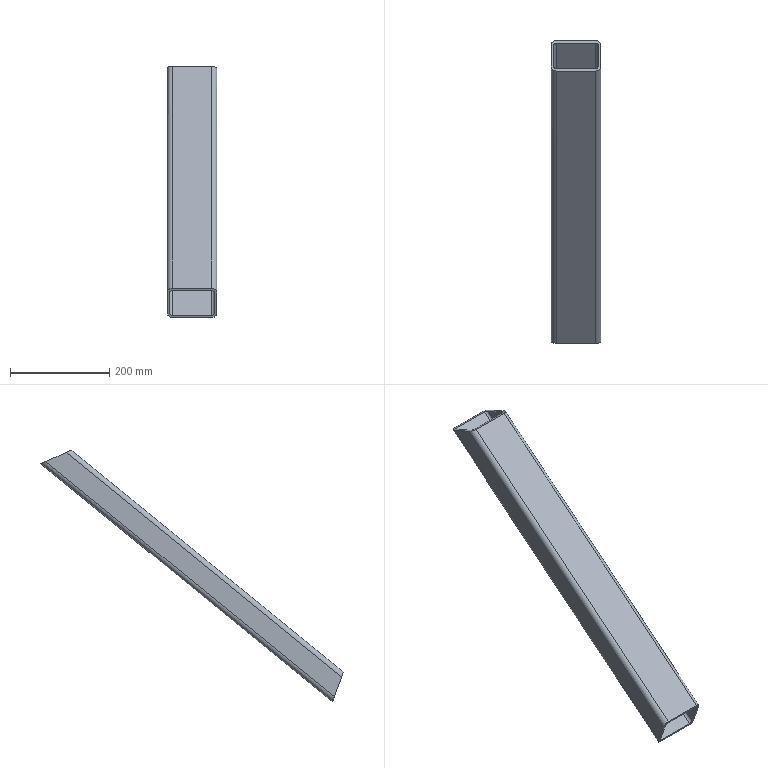Component | SolidWorks | Stap-1-10 | 1 solid | 18 faces | box 100 x 609.89 x 506.72 mm | volume 1052516 mm3 | plane 10 | cylinder 8 | commonest cylinder face diameters 20 x4 10 x4 | material Plain Carbon Steel
build123d program:
from build123d import *

# Parameters (mm, degrees)
BOSS_EXTRUDE1_DEPTH = 100
FILLET1_R           = 10
SHELL1_T            = -5


with BuildPart() as part:
    # Sketch1 → Boss-Extrude1 (new body)
    with BuildSketch(Plane.XY):
        Polygon((316.157, -65.741), (508.009, 668.488), (560.782, 633.12), (381.943, -51.308), align=None)
    extrude(amount=-BOSS_EXTRUDE1_DEPTH)

    # Fillet1
    fillet1_edges = [part.edges().sort_by_distance(p)[0] for p in [
        (412.083, 301.373, -100),
        (412.083, 301.373, 0),
        (471.362, 290.906, 0),
        (471.362, 290.906, -100),
    ]]
    fillet(fillet1_edges, radius=FILLET1_R)

    # Shell1
    shell1_openings = [part.faces().sort_by_distance(p)[0] for p in [
        (534.395, 650.804, -50),
        (349.05, -58.525, -50),
    ]]
    offset(amount=SHELL1_T, openings=shell1_openings, kind=Kind.INTERSECTION)


solid = part.part

# Placed as in the assembly
solid = solid.moved(Location((-734, -25.418, -30.778), (-126.164, 90, 0)))
STEP:
#1=COLOUR_RGB('',0.7922,0.8196,0.9333);
#2=FILL_AREA_STYLE_COLOUR('',#1);
#3=FILL_AREA_STYLE('',(#2));
#4=SURFACE_STYLE_FILL_AREA(#3);
#5=SURFACE_SIDE_STYLE('',(#4));
#6=SURFACE_STYLE_USAGE(.BOTH.,#5);
#7=PRESENTATION_STYLE_ASSIGNMENT((#6));
#8=CARTESIAN_POINT('',(-32.441,-9.522,8.223));
#9=VERTEX_POINT('',#8);
#10=CARTESIAN_POINT('',(-29.291,-9.522,8.223));
#11=VERTEX_POINT('',#10);
#12=CARTESIAN_POINT('',(-32.835,-9.522,8.223));
#13=DIRECTION('',(1.,-0.,0.));
#14=VECTOR('',#13,39.37);
#15=LINE('',#12,#14);
#16=EDGE_CURVE('',#9,#11,#15,.T.);
#17=ORIENTED_EDGE('',*,*,#16,.F.);
#18=CARTESIAN_POINT('',(-32.835,-9.927,8.401));
#19=VERTEX_POINT('',#18);
#20=CARTESIAN_POINT('',(-32.441,-9.522,8.223));
#21=CARTESIAN_POINT('',(-32.672,-9.522,8.223));
#22=CARTESIAN_POINT('',(-32.835,-9.69,8.297));
#23=CARTESIAN_POINT('',(-32.835,-9.927,8.401));
#24=(BOUNDED_CURVE()B_SPLINE_CURVE(3,(#20,#21,#22,#23),.UNSPECIFIED.,.F.,.T.)B_SPLINE_CURVE_WITH_KNOTS((4,4),(0.,1.571),.UNSPECIFIED.)CURVE()GEOMETRIC_REPRESENTATION_ITEM()RATIONAL_B_SPLINE_CURVE((1.,0.8047,0.8047,1.))REPRESENTATION_ITEM(''));
#25=EDGE_CURVE('',#9,#19,#24,.T.);
#26=ORIENTED_EDGE('',*,*,#25,.T.);
#27=CARTESIAN_POINT('',(-32.835,-11.544,9.114));
#28=VERTEX_POINT('',#27);
#29=CARTESIAN_POINT('',(-32.835,-11.949,9.292));
#30=DIRECTION('',(-0.,-0.915,0.4034));
#31=VECTOR('',#30,39.37);
#32=LINE('',#29,#31);
#33=EDGE_CURVE('',#19,#28,#32,.T.);
#34=ORIENTED_EDGE('',*,*,#33,.T.);
#35=CARTESIAN_POINT('',(-32.441,-11.949,9.292));
#36=VERTEX_POINT('',#35);
#37=CARTESIAN_POINT('',(-32.835,-11.544,9.114));
#38=CARTESIAN_POINT('',(-32.835,-11.781,9.219));
#39=CARTESIAN_POINT('',(-32.672,-11.949,9.292));
#40=CARTESIAN_POINT('',(-32.441,-11.949,9.292));
#41=(BOUNDED_CURVE()B_SPLINE_CURVE(3,(#37,#38,#39,#40),.UNSPECIFIED.,.F.,.T.)B_SPLINE_CURVE_WITH_KNOTS((4,4),(4.712,6.283),.UNSPECIFIED.)CURVE()GEOMETRIC_REPRESENTATION_ITEM()RATIONAL_B_SPLINE_CURVE((1.,0.8047,0.8047,1.))REPRESENTATION_ITEM(''));
#42=EDGE_CURVE('',#28,#36,#41,.T.);
#43=ORIENTED_EDGE('',*,*,#42,.T.);
#44=CARTESIAN_POINT('',(-29.291,-11.949,9.292));
#45=VERTEX_POINT('',#44);
#46=CARTESIAN_POINT('',(-32.835,-11.949,9.292));
#47=DIRECTION('',(1.,-0.,0.));
#48=VECTOR('',#47,39.37);
#49=LINE('',#46,#48);
#50=EDGE_CURVE('',#36,#45,#49,.T.);
#51=ORIENTED_EDGE('',*,*,#50,.T.);
#52=CARTESIAN_POINT('',(-28.898,-11.544,9.114));
#53=VERTEX_POINT('',#52);
#54=CARTESIAN_POINT('',(-29.291,-11.949,9.292));
#55=CARTESIAN_POINT('',(-29.061,-11.949,9.292));
#56=CARTESIAN_POINT('',(-28.898,-11.781,9.219));
#57=CARTESIAN_POINT('',(-28.898,-11.544,9.114));
#58=(BOUNDED_CURVE()B_SPLINE_CURVE(3,(#54,#55,#56,#57),.UNSPECIFIED.,.F.,.F.)B_SPLINE_CURVE_WITH_KNOTS((4,4),(3.142,4.712),.UNSPECIFIED.)CURVE()GEOMETRIC_REPRESENTATION_ITEM()RATIONAL_B_SPLINE_CURVE((1.,0.8047,0.8047,1.))REPRESENTATION_ITEM(''));
#59=EDGE_CURVE('',#45,#53,#58,.T.);
#60=ORIENTED_EDGE('',*,*,#59,.T.);
#61=CARTESIAN_POINT('',(-28.898,-9.927,8.401));
#62=VERTEX_POINT('',#61);
#63=CARTESIAN_POINT('',(-28.898,-11.949,9.292));
#64=DIRECTION('',(-0.,-0.915,0.4034));
#65=VECTOR('',#64,39.37);
#66=LINE('',#63,#65);
#67=EDGE_CURVE('',#62,#53,#66,.T.);
#68=ORIENTED_EDGE('',*,*,#67,.F.);
#69=CARTESIAN_POINT('',(-28.898,-9.927,8.401));
#70=CARTESIAN_POINT('',(-28.898,-9.69,8.297));
#71=CARTESIAN_POINT('',(-29.061,-9.522,8.223));
#72=CARTESIAN_POINT('',(-29.291,-9.522,8.223));
#73=(BOUNDED_CURVE()B_SPLINE_CURVE(3,(#69,#70,#71,#72),.UNSPECIFIED.,.F.,.T.)B_SPLINE_CURVE_WITH_KNOTS((4,4),(1.571,3.142),.UNSPECIFIED.)CURVE()GEOMETRIC_REPRESENTATION_ITEM()RATIONAL_B_SPLINE_CURVE((1.,0.8047,0.8047,1.))REPRESENTATION_ITEM(''));
#74=EDGE_CURVE('',#62,#11,#73,.T.);
#75=ORIENTED_EDGE('',*,*,#74,.T.);
#76=EDGE_LOOP('',(#17,#26,#34,#43,#51,#60,#68,#75));
#77=FACE_OUTER_BOUND('',#76,.T.);
#78=CARTESIAN_POINT('',(-32.441,-9.725,8.312));
#79=VERTEX_POINT('',#78);
#80=CARTESIAN_POINT('',(-32.638,-9.927,8.401));
#81=VERTEX_POINT('',#80);
#82=CARTESIAN_POINT('',(-32.441,-9.725,8.312));
#83=CARTESIAN_POINT('',(-32.556,-9.725,8.312));
#84=CARTESIAN_POINT('',(-32.638,-9.808,8.349));
#85=CARTESIAN_POINT('',(-32.638,-9.927,8.401));
#86=(BOUNDED_CURVE()B_SPLINE_CURVE(3,(#82,#83,#84,#85),.UNSPECIFIED.,.F.,.T.)B_SPLINE_CURVE_WITH_KNOTS((4,4),(0.,1.571),.UNSPECIFIED.)CURVE()GEOMETRIC_REPRESENTATION_ITEM()RATIONAL_B_SPLINE_CURVE((1.,0.8047,0.8047,1.))REPRESENTATION_ITEM(''));
#87=EDGE_CURVE('',#79,#81,#86,.T.);
#88=ORIENTED_EDGE('',*,*,#87,.F.);
#89=CARTESIAN_POINT('',(-29.291,-9.725,8.312));
#90=VERTEX_POINT('',#89);
#91=CARTESIAN_POINT('',(-32.835,-9.725,8.312));
#92=DIRECTION('',(1.,-0.,0.));
#93=VECTOR('',#92,39.37);
#94=LINE('',#91,#93);
#95=EDGE_CURVE('',#79,#90,#94,.T.);
#96=ORIENTED_EDGE('',*,*,#95,.T.);
#97=CARTESIAN_POINT('',(-29.094,-9.927,8.401));
#98=VERTEX_POINT('',#97);
#99=CARTESIAN_POINT('',(-29.094,-9.927,8.401));
#100=CARTESIAN_POINT('',(-29.094,-9.808,8.349));
#101=CARTESIAN_POINT('',(-29.176,-9.725,8.312));
#102=CARTESIAN_POINT('',(-29.291,-9.725,8.312));
#103=(BOUNDED_CURVE()B_SPLINE_CURVE(3,(#99,#100,#101,#102),.UNSPECIFIED.,.F.,.T.)B_SPLINE_CURVE_WITH_KNOTS((4,4),(1.571,3.142),.UNSPECIFIED.)CURVE()GEOMETRIC_REPRESENTATION_ITEM()RATIONAL_B_SPLINE_CURVE((1.,0.8047,0.8047,1.))REPRESENTATION_ITEM(''));
#104=EDGE_CURVE('',#98,#90,#103,.T.);
#105=ORIENTED_EDGE('',*,*,#104,.F.);
#106=CARTESIAN_POINT('',(-29.094,-11.544,9.114));
#107=VERTEX_POINT('',#106);
#108=CARTESIAN_POINT('',(-29.094,-11.949,9.292));
#109=DIRECTION('',(-0.,-0.915,0.4034));
#110=VECTOR('',#109,39.37);
#111=LINE('',#108,#110);
#112=EDGE_CURVE('',#98,#107,#111,.T.);
#113=ORIENTED_EDGE('',*,*,#112,.T.);
#114=CARTESIAN_POINT('',(-29.291,-11.746,9.203));
#115=VERTEX_POINT('',#114);
#116=CARTESIAN_POINT('',(-29.291,-11.746,9.203));
#117=CARTESIAN_POINT('',(-29.176,-11.746,9.203));
#118=CARTESIAN_POINT('',(-29.094,-11.663,9.166));
#119=CARTESIAN_POINT('',(-29.094,-11.544,9.114));
#120=(BOUNDED_CURVE()B_SPLINE_CURVE(3,(#116,#117,#118,#119),.UNSPECIFIED.,.F.,.T.)B_SPLINE_CURVE_WITH_KNOTS((4,4),(3.142,4.712),.UNSPECIFIED.)CURVE()GEOMETRIC_REPRESENTATION_ITEM()RATIONAL_B_SPLINE_CURVE((1.,0.8047,0.8047,1.))REPRESENTATION_ITEM(''));
#121=EDGE_CURVE('',#115,#107,#120,.T.);
#122=ORIENTED_EDGE('',*,*,#121,.F.);
#123=CARTESIAN_POINT('',(-32.441,-11.746,9.203));
#124=VERTEX_POINT('',#123);
#125=CARTESIAN_POINT('',(-32.835,-11.746,9.203));
#126=DIRECTION('',(1.,-0.,0.));
#127=VECTOR('',#126,39.37);
#128=LINE('',#125,#127);
#129=EDGE_CURVE('',#124,#115,#128,.T.);
#130=ORIENTED_EDGE('',*,*,#129,.F.);
#131=CARTESIAN_POINT('',(-32.638,-11.544,9.114));
#132=VERTEX_POINT('',#131);
#133=CARTESIAN_POINT('',(-32.638,-11.544,9.114));
#134=CARTESIAN_POINT('',(-32.638,-11.663,9.166));
#135=CARTESIAN_POINT('',(-32.556,-11.746,9.203));
#136=CARTESIAN_POINT('',(-32.441,-11.746,9.203));
#137=(BOUNDED_CURVE()B_SPLINE_CURVE(3,(#133,#134,#135,#136),.UNSPECIFIED.,.F.,.T.)B_SPLINE_CURVE_WITH_KNOTS((4,4),(4.712,6.283),.UNSPECIFIED.)CURVE()GEOMETRIC_REPRESENTATION_ITEM()RATIONAL_B_SPLINE_CURVE((1.,0.8047,0.8047,1.))REPRESENTATION_ITEM(''));
#138=EDGE_CURVE('',#132,#124,#137,.T.);
#139=ORIENTED_EDGE('',*,*,#138,.F.);
#140=CARTESIAN_POINT('',(-32.638,-11.949,9.292));
#141=DIRECTION('',(-0.,-0.915,0.4034));
#142=VECTOR('',#141,39.37);
#143=LINE('',#140,#142);
#144=EDGE_CURVE('',#81,#132,#143,.T.);
#145=ORIENTED_EDGE('',*,*,#144,.F.);
#146=EDGE_LOOP('',(#88,#96,#105,#113,#122,#130,#139,#145));
#147=FACE_BOUND('',#146,.T.);
#148=CARTESIAN_POINT('',(-32.835,-11.949,9.292));
#149=DIRECTION('',(-0.,0.4034,0.915));
#150=DIRECTION('',(-0.,-0.915,0.4034));
#151=AXIS2_PLACEMENT_3D('',#148,#149,#150);
#152=PLANE('',#151);
#153=ADVANCED_FACE('',(#77,#147),#152,.T.);
#154=CARTESIAN_POINT('',(-32.441,-32.678,-10.657));
#155=VERTEX_POINT('',#154);
#156=CARTESIAN_POINT('',(-29.291,-32.678,-10.657));
#157=VERTEX_POINT('',#156);
#158=CARTESIAN_POINT('',(-32.835,-32.678,-10.657));
#159=DIRECTION('',(1.,-0.,0.));
#160=VECTOR('',#159,39.37);
#161=LINE('',#158,#160);
#162=EDGE_CURVE('',#155,#157,#161,.T.);
#163=ORIENTED_EDGE('',*,*,#162,.F.);
#164=CARTESIAN_POINT('',(-32.441,-9.522,8.223));
#165=DIRECTION('',(-0.,0.775,0.6319));
#166=VECTOR('',#165,39.37);
#167=LINE('',#164,#166);
#168=EDGE_CURVE('',#155,#9,#167,.T.);
#169=ORIENTED_EDGE('',*,*,#168,.T.);
#170=ORIENTED_EDGE('',*,*,#16,.T.);
#171=CARTESIAN_POINT('',(-29.291,-32.678,-10.657));
#172=DIRECTION('',(0.,-0.775,-0.6319));
#173=VECTOR('',#172,39.37);
#174=LINE('',#171,#173);
#175=EDGE_CURVE('',#11,#157,#174,.T.);
#176=ORIENTED_EDGE('',*,*,#175,.T.);
#177=EDGE_LOOP('',(#163,#169,#170,#176));
#178=FACE_OUTER_BOUND('',#177,.T.);
#179=CARTESIAN_POINT('',(-32.835,-9.522,8.223));
#180=DIRECTION('',(0.,0.6319,-0.775));
#181=DIRECTION('',(-0.,0.775,0.6319));
#182=AXIS2_PLACEMENT_3D('',#179,#180,#181);
#183=PLANE('',#182);
#184=ADVANCED_FACE('',(#178),#183,.T.);
#185=CARTESIAN_POINT('',(-32.638,-33.391,-8.699));
#186=VERTEX_POINT('',#185);
#187=CARTESIAN_POINT('',(-32.638,-32.821,-10.266));
#188=VERTEX_POINT('',#187);
#189=CARTESIAN_POINT('',(-32.638,-32.678,-10.657));
#190=DIRECTION('',(0.,0.3421,-0.9397));
#191=VECTOR('',#190,39.37);
#192=LINE('',#189,#191);
#193=EDGE_CURVE('',#186,#188,#192,.T.);
#194=ORIENTED_EDGE('',*,*,#193,.F.);
#195=CARTESIAN_POINT('',(-32.441,-33.463,-8.503));
#196=VERTEX_POINT('',#195);
#197=CARTESIAN_POINT('',(-32.441,-33.463,-8.503));
#198=CARTESIAN_POINT('',(-32.556,-33.463,-8.503));
#199=CARTESIAN_POINT('',(-32.638,-33.433,-8.584));
#200=CARTESIAN_POINT('',(-32.638,-33.391,-8.699));
#201=(BOUNDED_CURVE()B_SPLINE_CURVE(3,(#197,#198,#199,#200),.UNSPECIFIED.,.F.,.T.)B_SPLINE_CURVE_WITH_KNOTS((4,4),(3.142,4.712),.UNSPECIFIED.)CURVE()GEOMETRIC_REPRESENTATION_ITEM()RATIONAL_B_SPLINE_CURVE((1.,0.8047,0.8047,1.))REPRESENTATION_ITEM(''));
#202=EDGE_CURVE('',#196,#186,#201,.T.);
#203=ORIENTED_EDGE('',*,*,#202,.F.);
#204=CARTESIAN_POINT('',(-29.291,-33.463,-8.503));
#205=VERTEX_POINT('',#204);
#206=CARTESIAN_POINT('',(-32.835,-33.463,-8.503));
#207=DIRECTION('',(1.,-0.,0.));
#208=VECTOR('',#207,39.37);
#209=LINE('',#206,#208);
#210=EDGE_CURVE('',#196,#205,#209,.T.);
#211=ORIENTED_EDGE('',*,*,#210,.T.);
#212=CARTESIAN_POINT('',(-29.094,-33.391,-8.699));
#213=VERTEX_POINT('',#212);
#214=CARTESIAN_POINT('',(-29.094,-33.391,-8.699));
#215=CARTESIAN_POINT('',(-29.094,-33.433,-8.584));
#216=CARTESIAN_POINT('',(-29.176,-33.463,-8.503));
#217=CARTESIAN_POINT('',(-29.291,-33.463,-8.503));
#218=(BOUNDED_CURVE()B_SPLINE_CURVE(3,(#214,#215,#216,#217),.UNSPECIFIED.,.F.,.T.)B_SPLINE_CURVE_WITH_KNOTS((4,4),(4.712,6.283),.UNSPECIFIED.)CURVE()GEOMETRIC_REPRESENTATION_ITEM()RATIONAL_B_SPLINE_CURVE((1.,0.8047,0.8047,1.))REPRESENTATION_ITEM(''));
#219=EDGE_CURVE('',#213,#205,#218,.T.);
#220=ORIENTED_EDGE('',*,*,#219,.F.);
#221=CARTESIAN_POINT('',(-29.094,-32.821,-10.266));
#222=VERTEX_POINT('',#221);
#223=CARTESIAN_POINT('',(-29.094,-32.678,-10.657));
#224=DIRECTION('',(0.,0.3421,-0.9397));
#225=VECTOR('',#224,39.37);
#226=LINE('',#223,#225);
#227=EDGE_CURVE('',#213,#222,#226,.T.);
#228=ORIENTED_EDGE('',*,*,#227,.T.);
#229=CARTESIAN_POINT('',(-29.291,-32.749,-10.461));
#230=VERTEX_POINT('',#229);
#231=CARTESIAN_POINT('',(-29.291,-32.749,-10.461));
#232=CARTESIAN_POINT('',(-29.176,-32.749,-10.461));
#233=CARTESIAN_POINT('',(-29.094,-32.779,-10.38));
#234=CARTESIAN_POINT('',(-29.094,-32.821,-10.266));
#235=(BOUNDED_CURVE()B_SPLINE_CURVE(3,(#231,#232,#233,#234),.UNSPECIFIED.,.F.,.T.)B_SPLINE_CURVE_WITH_KNOTS((4,4),(-0.,1.571),.UNSPECIFIED.)CURVE()GEOMETRIC_REPRESENTATION_ITEM()RATIONAL_B_SPLINE_CURVE((1.,0.8047,0.8047,1.))REPRESENTATION_ITEM(''));
#236=EDGE_CURVE('',#230,#222,#235,.T.);
#237=ORIENTED_EDGE('',*,*,#236,.F.);
#238=CARTESIAN_POINT('',(-32.441,-32.749,-10.461));
#239=VERTEX_POINT('',#238);
#240=CARTESIAN_POINT('',(-32.835,-32.749,-10.461));
#241=DIRECTION('',(1.,-0.,0.));
#242=VECTOR('',#241,39.37);
#243=LINE('',#240,#242);
#244=EDGE_CURVE('',#239,#230,#243,.T.);
#245=ORIENTED_EDGE('',*,*,#244,.F.);
#246=CARTESIAN_POINT('',(-32.638,-32.821,-10.266));
#247=CARTESIAN_POINT('',(-32.638,-32.779,-10.38));
#248=CARTESIAN_POINT('',(-32.556,-32.749,-10.461));
#249=CARTESIAN_POINT('',(-32.441,-32.749,-10.461));
#250=(BOUNDED_CURVE()B_SPLINE_CURVE(3,(#246,#247,#248,#249),.UNSPECIFIED.,.F.,.T.)B_SPLINE_CURVE_WITH_KNOTS((4,4),(1.571,3.142),.UNSPECIFIED.)CURVE()GEOMETRIC_REPRESENTATION_ITEM()RATIONAL_B_SPLINE_CURVE((1.,0.8047,0.8047,1.))REPRESENTATION_ITEM(''));
#251=EDGE_CURVE('',#188,#239,#250,.T.);
#252=ORIENTED_EDGE('',*,*,#251,.F.);
#253=EDGE_LOOP('',(#194,#203,#211,#220,#228,#237,#245,#252));
#254=FACE_BOUND('',#253,.T.);
#255=CARTESIAN_POINT('',(-32.835,-33.391,-8.699));
#256=VERTEX_POINT('',#255);
#257=CARTESIAN_POINT('',(-32.835,-32.821,-10.266));
#258=VERTEX_POINT('',#257);
#259=CARTESIAN_POINT('',(-32.835,-32.678,-10.657));
#260=DIRECTION('',(0.,0.3421,-0.9397));
#261=VECTOR('',#260,39.37);
#262=LINE('',#259,#261);
#263=EDGE_CURVE('',#256,#258,#262,.T.);
#264=ORIENTED_EDGE('',*,*,#263,.T.);
#265=CARTESIAN_POINT('',(-32.835,-32.821,-10.266));
#266=CARTESIAN_POINT('',(-32.835,-32.737,-10.495));
#267=CARTESIAN_POINT('',(-32.672,-32.678,-10.657));
#268=CARTESIAN_POINT('',(-32.441,-32.678,-10.657));
#269=(BOUNDED_CURVE()B_SPLINE_CURVE(3,(#265,#266,#267,#268),.UNSPECIFIED.,.F.,.T.)B_SPLINE_CURVE_WITH_KNOTS((4,4),(1.571,3.142),.UNSPECIFIED.)CURVE()GEOMETRIC_REPRESENTATION_ITEM()RATIONAL_B_SPLINE_CURVE((1.,0.8047,0.8047,1.))REPRESENTATION_ITEM(''));
#270=EDGE_CURVE('',#258,#155,#269,.T.);
#271=ORIENTED_EDGE('',*,*,#270,.T.);
#272=ORIENTED_EDGE('',*,*,#162,.T.);
#273=CARTESIAN_POINT('',(-28.898,-32.821,-10.266));
#274=VERTEX_POINT('',#273);
#275=CARTESIAN_POINT('',(-29.291,-32.678,-10.657));
#276=CARTESIAN_POINT('',(-29.061,-32.678,-10.657));
#277=CARTESIAN_POINT('',(-28.898,-32.737,-10.495));
#278=CARTESIAN_POINT('',(-28.898,-32.821,-10.266));
#279=(BOUNDED_CURVE()B_SPLINE_CURVE(3,(#275,#276,#277,#278),.UNSPECIFIED.,.F.,.T.)B_SPLINE_CURVE_WITH_KNOTS((4,4),(0.,1.571),.UNSPECIFIED.)CURVE()GEOMETRIC_REPRESENTATION_ITEM()RATIONAL_B_SPLINE_CURVE((1.,0.8047,0.8047,1.))REPRESENTATION_ITEM(''));
#280=EDGE_CURVE('',#157,#274,#279,.T.);
#281=ORIENTED_EDGE('',*,*,#280,.T.);
#282=CARTESIAN_POINT('',(-28.898,-33.391,-8.699));
#283=VERTEX_POINT('',#282);
#284=CARTESIAN_POINT('',(-28.898,-32.678,-10.657));
#285=DIRECTION('',(0.,0.3421,-0.9397));
#286=VECTOR('',#285,39.37);
#287=LINE('',#284,#286);
#288=EDGE_CURVE('',#283,#274,#287,.T.);
#289=ORIENTED_EDGE('',*,*,#288,.F.);
#290=CARTESIAN_POINT('',(-29.291,-33.534,-8.307));
#291=VERTEX_POINT('',#290);
#292=CARTESIAN_POINT('',(-28.898,-33.391,-8.699));
#293=CARTESIAN_POINT('',(-28.898,-33.475,-8.469));
#294=CARTESIAN_POINT('',(-29.061,-33.534,-8.307));
#295=CARTESIAN_POINT('',(-29.291,-33.534,-8.307));
#296=(BOUNDED_CURVE()B_SPLINE_CURVE(3,(#292,#293,#294,#295),.UNSPECIFIED.,.F.,.T.)B_SPLINE_CURVE_WITH_KNOTS((4,4),(4.712,6.283),.UNSPECIFIED.)CURVE()GEOMETRIC_REPRESENTATION_ITEM()RATIONAL_B_SPLINE_CURVE((1.,0.8047,0.8047,1.))REPRESENTATION_ITEM(''));
#297=EDGE_CURVE('',#283,#291,#296,.T.);
#298=ORIENTED_EDGE('',*,*,#297,.T.);
#299=CARTESIAN_POINT('',(-32.441,-33.534,-8.307));
#300=VERTEX_POINT('',#299);
#301=CARTESIAN_POINT('',(-32.835,-33.534,-8.307));
#302=DIRECTION('',(1.,-0.,0.));
#303=VECTOR('',#302,39.37);
#304=LINE('',#301,#303);
#305=EDGE_CURVE('',#300,#291,#304,.T.);
#306=ORIENTED_EDGE('',*,*,#305,.F.);
#307=CARTESIAN_POINT('',(-32.441,-33.534,-8.307));
#308=CARTESIAN_POINT('',(-32.672,-33.534,-8.307));
#309=CARTESIAN_POINT('',(-32.835,-33.475,-8.469));
#310=CARTESIAN_POINT('',(-32.835,-33.391,-8.699));
#311=(BOUNDED_CURVE()B_SPLINE_CURVE(3,(#307,#308,#309,#310),.UNSPECIFIED.,.F.,.T.)B_SPLINE_CURVE_WITH_KNOTS((4,4),(3.142,4.712),.UNSPECIFIED.)CURVE()GEOMETRIC_REPRESENTATION_ITEM()RATIONAL_B_SPLINE_CURVE((1.,0.8047,0.8047,1.))REPRESENTATION_ITEM(''));
#312=EDGE_CURVE('',#300,#256,#311,.T.);
#313=ORIENTED_EDGE('',*,*,#312,.T.);
#314=EDGE_LOOP('',(#264,#271,#272,#281,#289,#298,#306,#313));
#315=FACE_OUTER_BOUND('',#314,.T.);
#316=CARTESIAN_POINT('',(-32.835,-32.678,-10.657));
#317=DIRECTION('',(-0.,-0.9397,-0.3421));
#318=DIRECTION('',(0.,0.3421,-0.9397));
#319=AXIS2_PLACEMENT_3D('',#316,#317,#318);
#320=PLANE('',#319);
#321=ADVANCED_FACE('',(#254,#315),#320,.T.);
#322=ORIENTED_EDGE('',*,*,#50,.F.);
#323=CARTESIAN_POINT('',(-32.441,-33.534,-8.307));
#324=DIRECTION('',(0.,-0.775,-0.6319));
#325=VECTOR('',#324,39.37);
#326=LINE('',#323,#325);
#327=EDGE_CURVE('',#36,#300,#326,.T.);
#328=ORIENTED_EDGE('',*,*,#327,.T.);
#329=ORIENTED_EDGE('',*,*,#305,.T.);
#330=CARTESIAN_POINT('',(-29.291,-11.949,9.292));
#331=DIRECTION('',(-0.,0.775,0.6319));
#332=VECTOR('',#331,39.37);
#333=LINE('',#330,#332);
#334=EDGE_CURVE('',#291,#45,#333,.T.);
#335=ORIENTED_EDGE('',*,*,#334,.T.);
#336=EDGE_LOOP('',(#322,#328,#329,#335));
#337=FACE_OUTER_BOUND('',#336,.T.);
#338=CARTESIAN_POINT('',(-32.835,-33.534,-8.307));
#339=DIRECTION('',(-0.,-0.6319,0.775));
#340=DIRECTION('',(0.,-0.775,-0.6319));
#341=AXIS2_PLACEMENT_3D('',#338,#339,#340);
#342=PLANE('',#341);
#343=ADVANCED_FACE('',(#337),#342,.T.);
#344=ORIENTED_EDGE('',*,*,#33,.F.);
#345=CARTESIAN_POINT('',(-32.835,-9.273,8.934));
#346=DIRECTION('',(0.,-0.775,-0.6319));
#347=VECTOR('',#346,39.37);
#348=LINE('',#345,#347);
#349=EDGE_CURVE('',#19,#258,#348,.T.);
#350=ORIENTED_EDGE('',*,*,#349,.T.);
#351=ORIENTED_EDGE('',*,*,#263,.F.);
#352=CARTESIAN_POINT('',(-32.835,-10.268,10.155));
#353=DIRECTION('',(-0.,0.775,0.6319));
#354=VECTOR('',#353,39.37);
#355=LINE('',#352,#354);
#356=EDGE_CURVE('',#256,#28,#355,.T.);
#357=ORIENTED_EDGE('',*,*,#356,.T.);
#358=EDGE_LOOP('',(#344,#350,#351,#357));
#359=FACE_OUTER_BOUND('',#358,.T.);
#360=CARTESIAN_POINT('',(-32.835,-1.001,-1.212));
#361=DIRECTION('',(-1.,0.,-0.));
#362=DIRECTION('',(0.,0.8073,-0.5901));
#363=AXIS2_PLACEMENT_3D('',#360,#361,#362);
#364=PLANE('',#363);
#365=ADVANCED_FACE('',(#359),#364,.T.);
#366=ORIENTED_EDGE('',*,*,#288,.T.);
#367=CARTESIAN_POINT('',(-28.898,-9.771,8.528));
#368=DIRECTION('',(-0.,0.775,0.6319));
#369=VECTOR('',#368,39.37);
#370=LINE('',#367,#369);
#371=EDGE_CURVE('',#274,#62,#370,.T.);
#372=ORIENTED_EDGE('',*,*,#371,.T.);
#373=ORIENTED_EDGE('',*,*,#67,.T.);
#374=CARTESIAN_POINT('',(-28.898,-33.285,-8.612));
#375=DIRECTION('',(0.,-0.775,-0.6319));
#376=VECTOR('',#375,39.37);
#377=LINE('',#374,#376);
#378=EDGE_CURVE('',#53,#283,#377,.T.);
#379=ORIENTED_EDGE('',*,*,#378,.T.);
#380=EDGE_LOOP('',(#366,#372,#373,#379));
#381=FACE_OUTER_BOUND('',#380,.T.);
#382=CARTESIAN_POINT('',(-28.898,-1.001,-1.212));
#383=DIRECTION('',(-1.,0.,-0.));
#384=DIRECTION('',(0.,0.8073,-0.5901));
#385=AXIS2_PLACEMENT_3D('',#382,#383,#384);
#386=PLANE('',#385);
#387=ADVANCED_FACE('',(#381),#386,.F.);
#388=ORIENTED_EDGE('',*,*,#270,.F.);
#389=ORIENTED_EDGE('',*,*,#349,.F.);
#390=ORIENTED_EDGE('',*,*,#25,.F.);
#391=ORIENTED_EDGE('',*,*,#168,.F.);
#392=EDGE_LOOP('',(#388,#389,#390,#391));
#393=FACE_OUTER_BOUND('',#392,.T.);
#394=CARTESIAN_POINT('',(-32.441,-9.771,8.528));
#395=DIRECTION('',(-0.,0.775,0.6319));
#396=DIRECTION('',(0.,-0.6319,0.775));
#397=AXIS2_PLACEMENT_3D('',#394,#395,#396);
#398=CYLINDRICAL_SURFACE('',#397,0.3937);
#399=ADVANCED_FACE('',(#393),#398,.T.);
#400=ORIENTED_EDGE('',*,*,#42,.F.);
#401=ORIENTED_EDGE('',*,*,#356,.F.);
#402=ORIENTED_EDGE('',*,*,#312,.F.);
#403=ORIENTED_EDGE('',*,*,#327,.F.);
#404=EDGE_LOOP('',(#400,#401,#402,#403));
#405=FACE_OUTER_BOUND('',#404,.T.);
#406=CARTESIAN_POINT('',(-32.441,-33.285,-8.612));
#407=DIRECTION('',(0.,-0.775,-0.6319));
#408=DIRECTION('',(0.,0.6319,-0.775));
#409=AXIS2_PLACEMENT_3D('',#406,#407,#408);
#410=CYLINDRICAL_SURFACE('',#409,0.3937);
#411=ADVANCED_FACE('',(#405),#410,.T.);
#412=ORIENTED_EDGE('',*,*,#280,.F.);
#413=ORIENTED_EDGE('',*,*,#175,.F.);
#414=ORIENTED_EDGE('',*,*,#74,.F.);
#415=ORIENTED_EDGE('',*,*,#371,.F.);
#416=EDGE_LOOP('',(#412,#413,#414,#415));
#417=FACE_OUTER_BOUND('',#416,.T.);
#418=CARTESIAN_POINT('',(-29.291,-9.273,8.934));
#419=DIRECTION('',(0.,-0.775,-0.6319));
#420=DIRECTION('',(0.,0.6319,-0.775));
#421=AXIS2_PLACEMENT_3D('',#418,#419,#420);
#422=CYLINDRICAL_SURFACE('',#421,0.3937);
#423=ADVANCED_FACE('',(#417),#422,.T.);
#424=ORIENTED_EDGE('',*,*,#59,.F.);
#425=ORIENTED_EDGE('',*,*,#334,.F.);
#426=ORIENTED_EDGE('',*,*,#297,.F.);
#427=ORIENTED_EDGE('',*,*,#378,.F.);
#428=EDGE_LOOP('',(#424,#425,#426,#427));
#429=FACE_OUTER_BOUND('',#428,.T.);
#430=CARTESIAN_POINT('',(-29.291,-10.268,10.155));
#431=DIRECTION('',(-0.,0.775,0.6319));
#432=DIRECTION('',(0.,-0.6319,0.775));
#433=AXIS2_PLACEMENT_3D('',#430,#431,#432);
#434=CYLINDRICAL_SURFACE('',#433,0.3937);
#435=ADVANCED_FACE('',(#429),#434,.T.);
#436=ORIENTED_EDGE('',*,*,#244,.T.);
#437=CARTESIAN_POINT('',(-29.291,-9.647,8.375));
#438=DIRECTION('',(0.,-0.775,-0.6319));
#439=VECTOR('',#438,39.37);
#440=LINE('',#437,#439);
#441=EDGE_CURVE('',#90,#230,#440,.T.);
#442=ORIENTED_EDGE('',*,*,#441,.F.);
#443=ORIENTED_EDGE('',*,*,#95,.F.);
#444=CARTESIAN_POINT('',(-32.441,-9.647,8.375));
#445=DIRECTION('',(-0.,0.775,0.6319));
#446=VECTOR('',#445,39.37);
#447=LINE('',#444,#446);
#448=EDGE_CURVE('',#239,#79,#447,.T.);
#449=ORIENTED_EDGE('',*,*,#448,.F.);
#450=EDGE_LOOP('',(#436,#442,#443,#449));
#451=FACE_OUTER_BOUND('',#450,.T.);
#452=CARTESIAN_POINT('',(-32.835,-9.647,8.375));
#453=DIRECTION('',(0.,0.6319,-0.775));
#454=DIRECTION('',(-0.,0.775,0.6319));
#455=AXIS2_PLACEMENT_3D('',#452,#453,#454);
#456=PLANE('',#455);
#457=ADVANCED_FACE('',(#451),#456,.F.);
#458=ORIENTED_EDGE('',*,*,#129,.T.);
#459=CARTESIAN_POINT('',(-29.291,-33.409,-8.46));
#460=DIRECTION('',(-0.,0.775,0.6319));
#461=VECTOR('',#460,39.37);
#462=LINE('',#459,#461);
#463=EDGE_CURVE('',#205,#115,#462,.T.);
#464=ORIENTED_EDGE('',*,*,#463,.F.);
#465=ORIENTED_EDGE('',*,*,#210,.F.);
#466=CARTESIAN_POINT('',(-32.441,-33.409,-8.46));
#467=DIRECTION('',(0.,-0.775,-0.6319));
#468=VECTOR('',#467,39.37);
#469=LINE('',#466,#468);
#470=EDGE_CURVE('',#124,#196,#469,.T.);
#471=ORIENTED_EDGE('',*,*,#470,.F.);
#472=EDGE_LOOP('',(#458,#464,#465,#471));
#473=FACE_OUTER_BOUND('',#472,.T.);
#474=CARTESIAN_POINT('',(-32.835,-33.409,-8.46));
#475=DIRECTION('',(-0.,-0.6319,0.775));
#476=DIRECTION('',(0.,-0.775,-0.6319));
#477=AXIS2_PLACEMENT_3D('',#474,#475,#476);
#478=PLANE('',#477);
#479=ADVANCED_FACE('',(#473),#478,.F.);
#480=ORIENTED_EDGE('',*,*,#144,.T.);
#481=CARTESIAN_POINT('',(-32.638,-33.285,-8.612));
#482=DIRECTION('',(-0.,0.775,0.6319));
#483=VECTOR('',#482,39.37);
#484=LINE('',#481,#483);
#485=EDGE_CURVE('',#186,#132,#484,.T.);
#486=ORIENTED_EDGE('',*,*,#485,.F.);
#487=ORIENTED_EDGE('',*,*,#193,.T.);
#488=CARTESIAN_POINT('',(-32.638,-9.771,8.528));
#489=DIRECTION('',(0.,-0.775,-0.6319));
#490=VECTOR('',#489,39.37);
#491=LINE('',#488,#490);
#492=EDGE_CURVE('',#81,#188,#491,.T.);
#493=ORIENTED_EDGE('',*,*,#492,.F.);
#494=EDGE_LOOP('',(#480,#486,#487,#493));
#495=FACE_OUTER_BOUND('',#494,.T.);
#496=CARTESIAN_POINT('',(-32.638,-1.001,-1.212));
#497=DIRECTION('',(-1.,0.,-0.));
#498=DIRECTION('',(0.,0.8073,-0.5901));
#499=AXIS2_PLACEMENT_3D('',#496,#497,#498);
#500=PLANE('',#499);
#501=ADVANCED_FACE('',(#495),#500,.F.);
#502=ORIENTED_EDGE('',*,*,#227,.F.);
#503=CARTESIAN_POINT('',(-29.094,-10.268,10.155));
#504=DIRECTION('',(0.,-0.775,-0.6319));
#505=VECTOR('',#504,39.37);
#506=LINE('',#503,#505);
#507=EDGE_CURVE('',#107,#213,#506,.T.);
#508=ORIENTED_EDGE('',*,*,#507,.F.);
#509=ORIENTED_EDGE('',*,*,#112,.F.);
#510=CARTESIAN_POINT('',(-29.094,-9.273,8.934));
#511=DIRECTION('',(-0.,0.775,0.6319));
#512=VECTOR('',#511,39.37);
#513=LINE('',#510,#512);
#514=EDGE_CURVE('',#222,#98,#513,.T.);
#515=ORIENTED_EDGE('',*,*,#514,.F.);
#516=EDGE_LOOP('',(#502,#508,#509,#515));
#517=FACE_OUTER_BOUND('',#516,.T.);
#518=CARTESIAN_POINT('',(-29.094,-1.001,-1.212));
#519=DIRECTION('',(-1.,0.,-0.));
#520=DIRECTION('',(0.,0.8073,-0.5901));
#521=AXIS2_PLACEMENT_3D('',#518,#519,#520);
#522=PLANE('',#521);
#523=ADVANCED_FACE('',(#517),#522,.T.);
#524=ORIENTED_EDGE('',*,*,#251,.T.);
#525=ORIENTED_EDGE('',*,*,#448,.T.);
#526=ORIENTED_EDGE('',*,*,#87,.T.);
#527=ORIENTED_EDGE('',*,*,#492,.T.);
#528=EDGE_LOOP('',(#524,#525,#526,#527));
#529=FACE_OUTER_BOUND('',#528,.T.);
#530=CARTESIAN_POINT('',(-32.441,-9.771,8.528));
#531=DIRECTION('',(-0.,0.775,0.6319));
#532=DIRECTION('',(0.,-0.6319,0.775));
#533=AXIS2_PLACEMENT_3D('',#530,#531,#532);
#534=CYLINDRICAL_SURFACE('',#533,0.1969);
#535=ADVANCED_FACE('',(#529),#534,.F.);
#536=ORIENTED_EDGE('',*,*,#138,.T.);
#537=ORIENTED_EDGE('',*,*,#470,.T.);
#538=ORIENTED_EDGE('',*,*,#202,.T.);
#539=ORIENTED_EDGE('',*,*,#485,.T.);
#540=EDGE_LOOP('',(#536,#537,#538,#539));
#541=FACE_OUTER_BOUND('',#540,.T.);
#542=CARTESIAN_POINT('',(-32.441,-33.285,-8.612));
#543=DIRECTION('',(0.,-0.775,-0.6319));
#544=DIRECTION('',(0.,0.6319,-0.775));
#545=AXIS2_PLACEMENT_3D('',#542,#543,#544);
#546=CYLINDRICAL_SURFACE('',#545,0.1969);
#547=ADVANCED_FACE('',(#541),#546,.F.);
#548=ORIENTED_EDGE('',*,*,#236,.T.);
#549=ORIENTED_EDGE('',*,*,#514,.T.);
#550=ORIENTED_EDGE('',*,*,#104,.T.);
#551=ORIENTED_EDGE('',*,*,#441,.T.);
#552=EDGE_LOOP('',(#548,#549,#550,#551));
#553=FACE_OUTER_BOUND('',#552,.T.);
#554=CARTESIAN_POINT('',(-29.291,-9.273,8.934));
#555=DIRECTION('',(0.,-0.775,-0.6319));
#556=DIRECTION('',(0.,0.6319,-0.775));
#557=AXIS2_PLACEMENT_3D('',#554,#555,#556);
#558=CYLINDRICAL_SURFACE('',#557,0.1969);
#559=ADVANCED_FACE('',(#553),#558,.F.);
#560=ORIENTED_EDGE('',*,*,#121,.T.);
#561=ORIENTED_EDGE('',*,*,#507,.T.);
#562=ORIENTED_EDGE('',*,*,#219,.T.);
#563=ORIENTED_EDGE('',*,*,#463,.T.);
#564=EDGE_LOOP('',(#560,#561,#562,#563));
#565=FACE_OUTER_BOUND('',#564,.T.);
#566=CARTESIAN_POINT('',(-29.291,-10.268,10.155));
#567=DIRECTION('',(-0.,0.775,0.6319));
#568=DIRECTION('',(0.,-0.6319,0.775));
#569=AXIS2_PLACEMENT_3D('',#566,#567,#568);
#570=CYLINDRICAL_SURFACE('',#569,0.1969);
#571=ADVANCED_FACE('',(#565),#570,.F.);
#572=CLOSED_SHELL('',(#153,#184,#321,#343,#365,#387,#399,#411,#423,#435,#457,#479,#501,#523,#535,#547,#559,#571));
#573=MANIFOLD_SOLID_BREP('',#572);
#574=STYLED_ITEM('',(#7),#573);
#575=PRESENTATION_LAYER_ASSIGNMENT('','',(#574));
#576=(LENGTH_UNIT()NAMED_UNIT(*)SI_UNIT($,.METRE.));
#577=LENGTH_MEASURE_WITH_UNIT(LENGTH_MEASURE(0.0254),#576);
#578=DIMENSIONAL_EXPONENTS(1.,0.,0.,0.,0.,0.,0.);
#579=(CONVERSION_BASED_UNIT('',#577)LENGTH_UNIT()NAMED_UNIT(#578));
#580=UNCERTAINTY_MEASURE_WITH_UNIT(LENGTH_MEASURE(0.00001),#579,'','');
#581=(NAMED_UNIT(*)PLANE_ANGLE_UNIT()SI_UNIT($,.RADIAN.));
#582=(NAMED_UNIT(*)SI_UNIT($,.STERADIAN.)SOLID_ANGLE_UNIT());
#583=(GEOMETRIC_REPRESENTATION_CONTEXT(3)GLOBAL_UNCERTAINTY_ASSIGNED_CONTEXT((#580))GLOBAL_UNIT_ASSIGNED_CONTEXT((#579,#581,#582))REPRESENTATION_CONTEXT('',''));
#584=MECHANICAL_DESIGN_GEOMETRIC_PRESENTATION_REPRESENTATION('',(#574),#583);
#585=CARTESIAN_POINT('',(0.,0.,0.));
#586=DIRECTION('',(0.,0.,1.));
#587=DIRECTION('',(1.,0.,0.));
#588=AXIS2_PLACEMENT_3D('',#585,#586,#587);
#589=(LENGTH_UNIT()NAMED_UNIT(*)SI_UNIT($,.METRE.));
#590=LENGTH_MEASURE_WITH_UNIT(LENGTH_MEASURE(0.0254),#589);
#591=DIMENSIONAL_EXPONENTS(1.,0.,0.,0.,0.,0.,0.);
#592=(CONVERSION_BASED_UNIT('',#590)LENGTH_UNIT()NAMED_UNIT(#591));
#593=UNCERTAINTY_MEASURE_WITH_UNIT(LENGTH_MEASURE(0.00001),#592,'','');
#594=(NAMED_UNIT(*)PLANE_ANGLE_UNIT()SI_UNIT($,.RADIAN.));
#595=(NAMED_UNIT(*)SI_UNIT($,.STERADIAN.)SOLID_ANGLE_UNIT());
#596=(GEOMETRIC_REPRESENTATION_CONTEXT(3)GLOBAL_UNCERTAINTY_ASSIGNED_CONTEXT((#593))GLOBAL_UNIT_ASSIGNED_CONTEXT((#592,#594,#595))REPRESENTATION_CONTEXT('',''));
#597=ADVANCED_BREP_SHAPE_REPRESENTATION('',(#573,#588),#596);